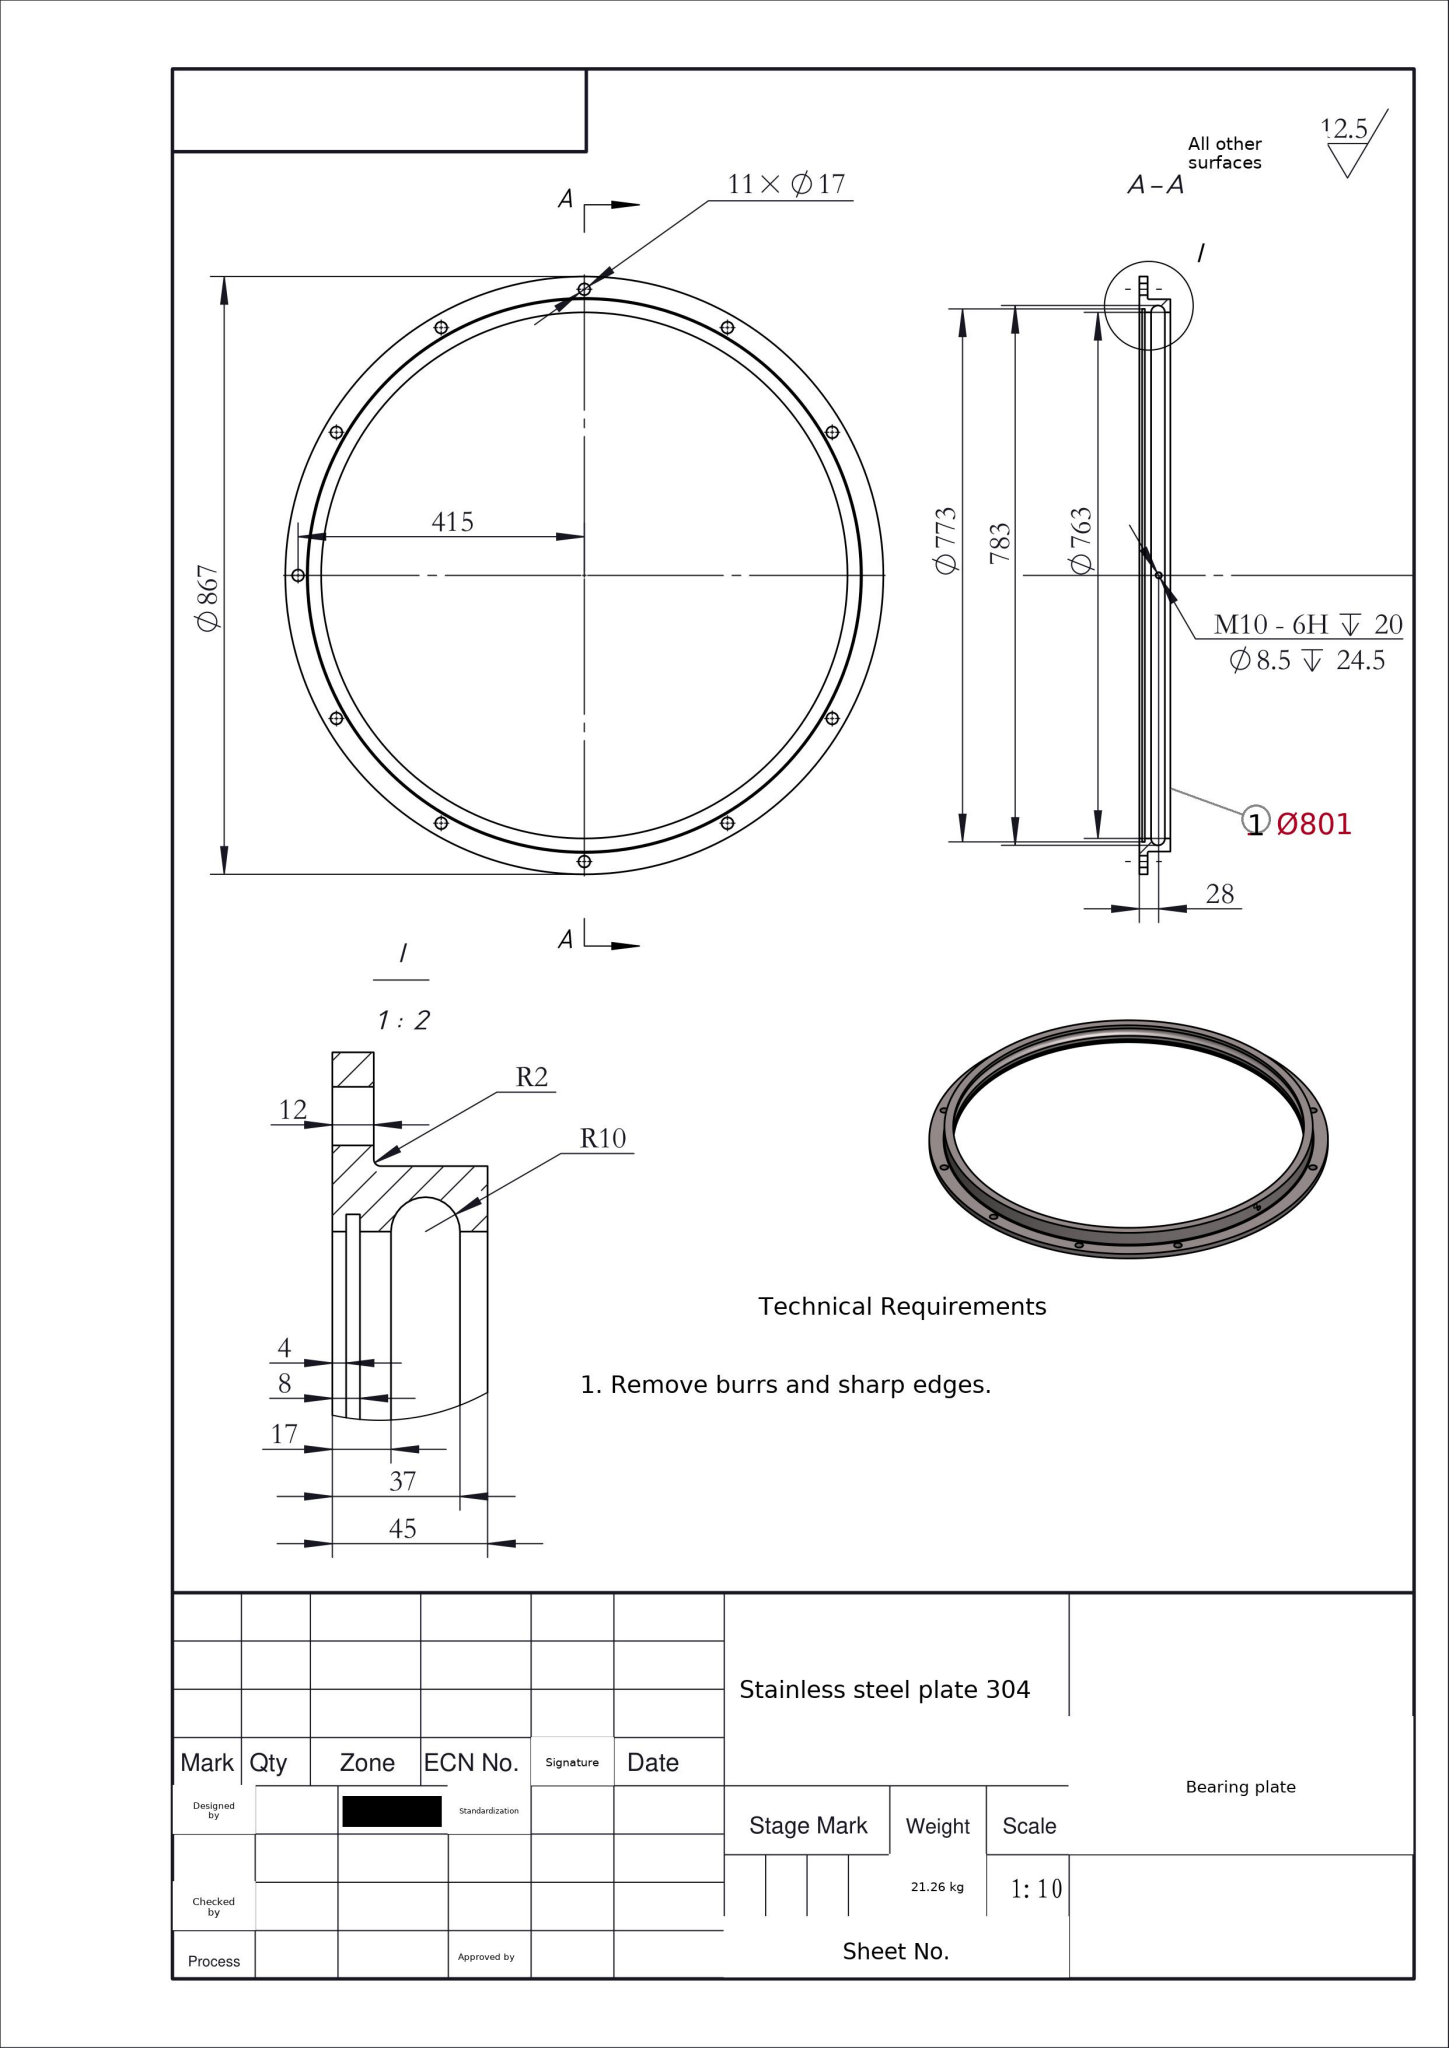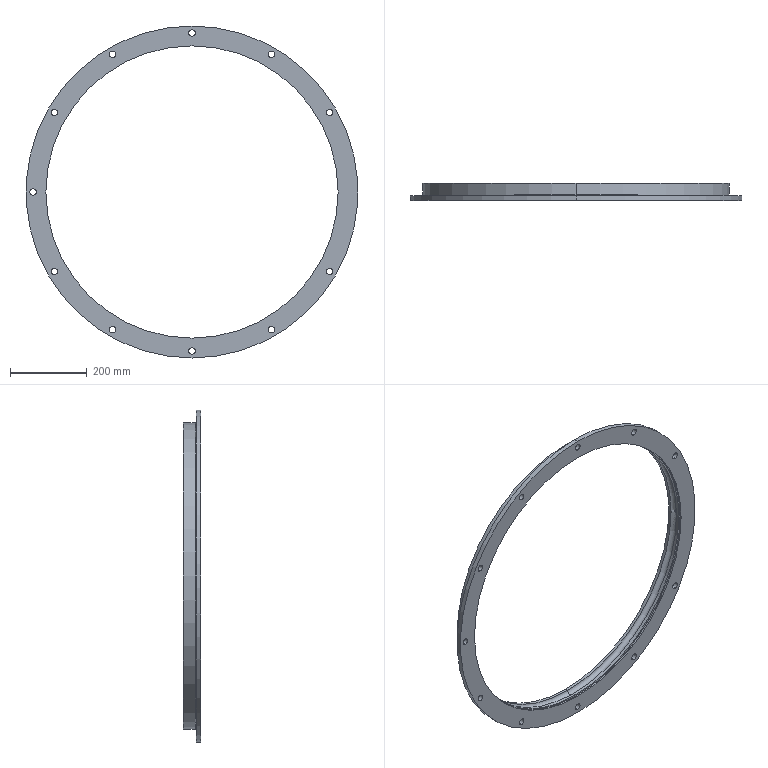Part | SolidWorks | mm | material Stainless steel plate 304 | 1 solid | 45 faces | box 867 x 45 x 867 mm | volume 2680761 mm3 | cylinder 36 | plane 5 | torus 4 | commonest cylinder face diameters 17 x22 763 x6 8.5 x2 867 x2 801 x2 773 x2